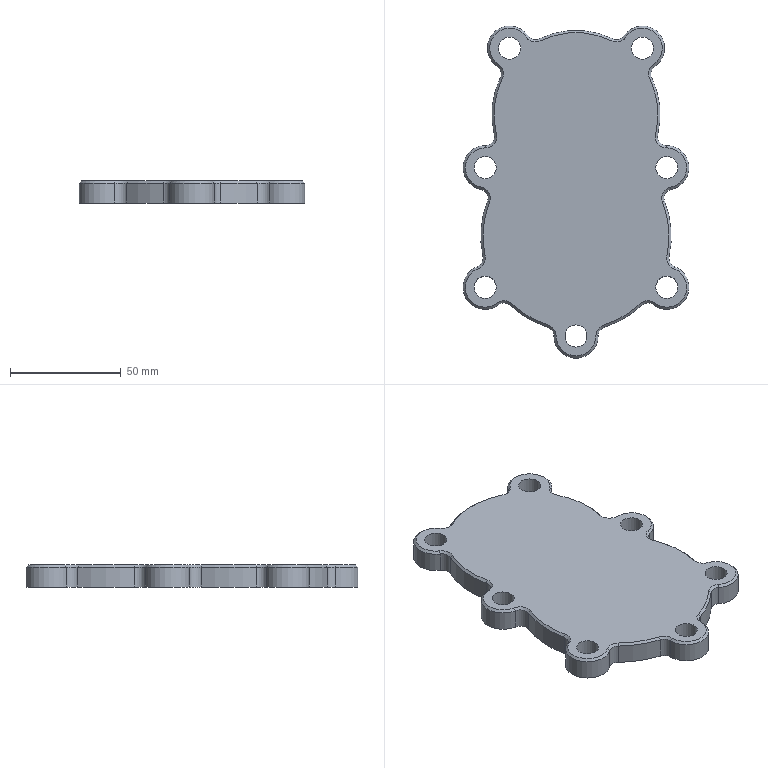Component | NX | 2_SIDE_COVER | 1 solid | 65 faces | volume 105650 mm3 | cylinder 35 | cone 28 | plane 2 | commonest cylinder face diameters 8 x14 20 x7 10 x7 86 x4 76 x3